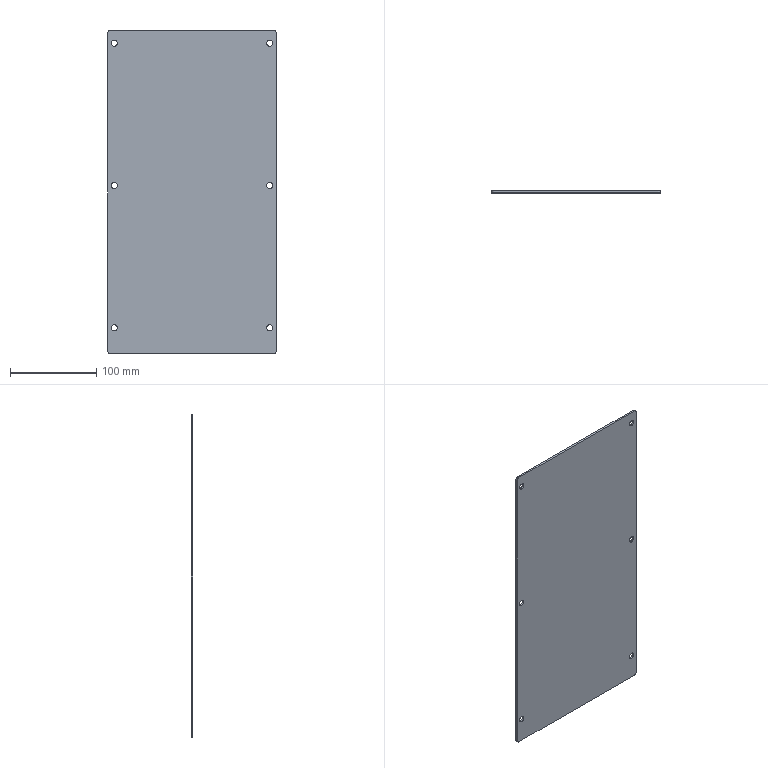Component | SolidWorks | CoverPlate4-1 | 1 solid | 22 faces | box 195 x 2 x 375 mm | volume 145773 mm3 | cylinder 16 | plane 6 | commonest cylinder face diameters 7 x12 6 x4 | material Plain Carbon Steel
build123d program:
from build123d import *

# Parameters (mm, degrees)
SKETCH1_W           = 375
SKETCH1_H           = 195
BOSS_EXTRUDE1_DEPTH = 2
SKETCH2_R           = 3.5
CUT_EXTRUDE1_DEPTH  = 2
FILLET1_R           = 3


with BuildPart() as part:
    # Sketch1 → Boss-Extrude1 (new body)
    with BuildSketch(Plane.XY):
        Rectangle(SKETCH1_W, SKETCH1_H)
    extrude(amount=BOSS_EXTRUDE1_DEPTH)

    # Sketch2 → Cut-Extrude1 (cut)
    with BuildSketch(Plane.XY.offset(2)):
        with Locations((-172.5, 90)):
            Circle(SKETCH2_R)
        with Locations((-7.5, 90)):
            Circle(SKETCH2_R)
        with Locations((-7.5, -90)):
            Circle(SKETCH2_R)
        with Locations((-172.5, -90)):
            Circle(SKETCH2_R)
        with Locations((157.5, 90)):
            Circle(SKETCH2_R)
        with Locations((157.5, -90)):
            Circle(SKETCH2_R)
    extrude(amount=-CUT_EXTRUDE1_DEPTH, mode=Mode.SUBTRACT)

    # Fillet1
    fillet1_edges = [part.edges().sort_by_distance(p)[0] for p in [
        (-187.5, 97.5, 1),
        (187.5, 97.5, 1),
        (187.5, -97.5, 1),
        (-187.5, -97.5, 1),
    ]]
    fillet(fillet1_edges, radius=FILLET1_R)


solid = part.part

# Placed as in the assembly
solid = solid.moved(Location((-47.166, -39.736, 10), (90, 0, -90)))
STEP:
#1=COLOUR_RGB('',0.7922,0.8196,0.9333);
#2=FILL_AREA_STYLE_COLOUR('',#1);
#3=FILL_AREA_STYLE('',(#2));
#4=SURFACE_STYLE_FILL_AREA(#3);
#5=SURFACE_SIDE_STYLE('',(#4));
#6=SURFACE_STYLE_USAGE(.BOTH.,#5);
#7=PRESENTATION_STYLE_ASSIGNMENT((#6));
#8=CARTESIAN_POINT('',(-5.4,-1.564,-5.669));
#9=VERTEX_POINT('',#8);
#10=CARTESIAN_POINT('',(-5.4,-1.564,-5.945));
#11=VERTEX_POINT('',#10);
#12=CARTESIAN_POINT('',(-5.4,-1.564,-5.807));
#13=DIRECTION('',(-0.,-1.,0.));
#14=DIRECTION('',(0.,0.,-1.));
#15=AXIS2_PLACEMENT_3D('',#12,#13,#14);
#16=CIRCLE('',#15,0.1378);
#17=EDGE_CURVE('',#9,#11,#16,.T.);
#18=ORIENTED_EDGE('',*,*,#17,.F.);
#19=CARTESIAN_POINT('',(-5.4,-1.643,-5.669));
#20=VERTEX_POINT('',#19);
#21=CARTESIAN_POINT('',(-5.4,-1.564,-5.669));
#22=DIRECTION('',(-0.,-1.,0.));
#23=VECTOR('',#22,39.37);
#24=LINE('',#21,#23);
#25=EDGE_CURVE('',#9,#20,#24,.T.);
#26=ORIENTED_EDGE('',*,*,#25,.T.);
#27=CARTESIAN_POINT('',(-5.4,-1.643,-5.945));
#28=VERTEX_POINT('',#27);
#29=CARTESIAN_POINT('',(-5.4,-1.643,-5.807));
#30=DIRECTION('',(-0.,-1.,0.));
#31=DIRECTION('',(0.,0.,-1.));
#32=AXIS2_PLACEMENT_3D('',#29,#30,#31);
#33=CIRCLE('',#32,0.1378);
#34=EDGE_CURVE('',#20,#28,#33,.T.);
#35=ORIENTED_EDGE('',*,*,#34,.T.);
#36=CARTESIAN_POINT('',(-5.4,-1.564,-5.945));
#37=DIRECTION('',(-0.,-1.,0.));
#38=VECTOR('',#37,39.37);
#39=LINE('',#36,#38);
#40=EDGE_CURVE('',#11,#28,#39,.T.);
#41=ORIENTED_EDGE('',*,*,#40,.F.);
#42=EDGE_LOOP('',(#18,#26,#35,#41));
#43=FACE_OUTER_BOUND('',#42,.T.);
#44=CARTESIAN_POINT('',(-5.4,-1.564,-5.807));
#45=DIRECTION('',(-0.,-1.,0.));
#46=DIRECTION('',(0.,0.,-1.));
#47=AXIS2_PLACEMENT_3D('',#44,#45,#46);
#48=CYLINDRICAL_SURFACE('',#47,0.1378);
#49=ADVANCED_FACE('',(#43),#48,.F.);
#50=CARTESIAN_POINT('',(1.686,-1.564,-5.669));
#51=VERTEX_POINT('',#50);
#52=CARTESIAN_POINT('',(1.686,-1.564,-5.945));
#53=VERTEX_POINT('',#52);
#54=CARTESIAN_POINT('',(1.686,-1.564,-5.807));
#55=DIRECTION('',(-0.,-1.,0.));
#56=DIRECTION('',(0.,0.,-1.));
#57=AXIS2_PLACEMENT_3D('',#54,#55,#56);
#58=CIRCLE('',#57,0.1378);
#59=EDGE_CURVE('',#51,#53,#58,.T.);
#60=ORIENTED_EDGE('',*,*,#59,.F.);
#61=CARTESIAN_POINT('',(1.686,-1.643,-5.669));
#62=VERTEX_POINT('',#61);
#63=CARTESIAN_POINT('',(1.686,-1.564,-5.669));
#64=DIRECTION('',(-0.,-1.,0.));
#65=VECTOR('',#64,39.37);
#66=LINE('',#63,#65);
#67=EDGE_CURVE('',#51,#62,#66,.T.);
#68=ORIENTED_EDGE('',*,*,#67,.T.);
#69=CARTESIAN_POINT('',(1.686,-1.643,-5.945));
#70=VERTEX_POINT('',#69);
#71=CARTESIAN_POINT('',(1.686,-1.643,-5.807));
#72=DIRECTION('',(-0.,-1.,0.));
#73=DIRECTION('',(0.,0.,-1.));
#74=AXIS2_PLACEMENT_3D('',#71,#72,#73);
#75=CIRCLE('',#74,0.1378);
#76=EDGE_CURVE('',#62,#70,#75,.T.);
#77=ORIENTED_EDGE('',*,*,#76,.T.);
#78=CARTESIAN_POINT('',(1.686,-1.564,-5.945));
#79=DIRECTION('',(-0.,-1.,0.));
#80=VECTOR('',#79,39.37);
#81=LINE('',#78,#80);
#82=EDGE_CURVE('',#53,#70,#81,.T.);
#83=ORIENTED_EDGE('',*,*,#82,.F.);
#84=EDGE_LOOP('',(#60,#68,#77,#83));
#85=FACE_OUTER_BOUND('',#84,.T.);
#86=CARTESIAN_POINT('',(1.686,-1.564,-5.807));
#87=DIRECTION('',(-0.,-1.,0.));
#88=DIRECTION('',(0.,0.,-1.));
#89=AXIS2_PLACEMENT_3D('',#86,#87,#88);
#90=CYLINDRICAL_SURFACE('',#89,0.1378);
#91=ADVANCED_FACE('',(#85),#90,.F.);
#92=CARTESIAN_POINT('',(-5.4,-1.564,7.323));
#93=VERTEX_POINT('',#92);
#94=CARTESIAN_POINT('',(-5.4,-1.564,7.047));
#95=VERTEX_POINT('',#94);
#96=CARTESIAN_POINT('',(-5.4,-1.564,7.185));
#97=DIRECTION('',(-0.,-1.,0.));
#98=DIRECTION('',(0.,0.,-1.));
#99=AXIS2_PLACEMENT_3D('',#96,#97,#98);
#100=CIRCLE('',#99,0.1378);
#101=EDGE_CURVE('',#93,#95,#100,.T.);
#102=ORIENTED_EDGE('',*,*,#101,.F.);
#103=CARTESIAN_POINT('',(-5.4,-1.643,7.323));
#104=VERTEX_POINT('',#103);
#105=CARTESIAN_POINT('',(-5.4,-1.564,7.323));
#106=DIRECTION('',(-0.,-1.,0.));
#107=VECTOR('',#106,39.37);
#108=LINE('',#105,#107);
#109=EDGE_CURVE('',#93,#104,#108,.T.);
#110=ORIENTED_EDGE('',*,*,#109,.T.);
#111=CARTESIAN_POINT('',(-5.4,-1.643,7.047));
#112=VERTEX_POINT('',#111);
#113=CARTESIAN_POINT('',(-5.4,-1.643,7.185));
#114=DIRECTION('',(-0.,-1.,0.));
#115=DIRECTION('',(0.,0.,-1.));
#116=AXIS2_PLACEMENT_3D('',#113,#114,#115);
#117=CIRCLE('',#116,0.1378);
#118=EDGE_CURVE('',#104,#112,#117,.T.);
#119=ORIENTED_EDGE('',*,*,#118,.T.);
#120=CARTESIAN_POINT('',(-5.4,-1.564,7.047));
#121=DIRECTION('',(-0.,-1.,0.));
#122=VECTOR('',#121,39.37);
#123=LINE('',#120,#122);
#124=EDGE_CURVE('',#95,#112,#123,.T.);
#125=ORIENTED_EDGE('',*,*,#124,.F.);
#126=EDGE_LOOP('',(#102,#110,#119,#125));
#127=FACE_OUTER_BOUND('',#126,.T.);
#128=CARTESIAN_POINT('',(-5.4,-1.564,7.185));
#129=DIRECTION('',(-0.,-1.,0.));
#130=DIRECTION('',(0.,0.,-1.));
#131=AXIS2_PLACEMENT_3D('',#128,#129,#130);
#132=CYLINDRICAL_SURFACE('',#131,0.1378);
#133=ADVANCED_FACE('',(#127),#132,.F.);
#134=CARTESIAN_POINT('',(-5.4,-1.564,0.8268));
#135=VERTEX_POINT('',#134);
#136=CARTESIAN_POINT('',(-5.4,-1.564,0.5512));
#137=VERTEX_POINT('',#136);
#138=CARTESIAN_POINT('',(-5.4,-1.564,0.689));
#139=DIRECTION('',(-0.,-1.,0.));
#140=DIRECTION('',(0.,0.,-1.));
#141=AXIS2_PLACEMENT_3D('',#138,#139,#140);
#142=CIRCLE('',#141,0.1378);
#143=EDGE_CURVE('',#135,#137,#142,.T.);
#144=ORIENTED_EDGE('',*,*,#143,.F.);
#145=CARTESIAN_POINT('',(-5.4,-1.643,0.8268));
#146=VERTEX_POINT('',#145);
#147=CARTESIAN_POINT('',(-5.4,-1.564,0.8268));
#148=DIRECTION('',(-0.,-1.,0.));
#149=VECTOR('',#148,39.37);
#150=LINE('',#147,#149);
#151=EDGE_CURVE('',#135,#146,#150,.T.);
#152=ORIENTED_EDGE('',*,*,#151,.T.);
#153=CARTESIAN_POINT('',(-5.4,-1.643,0.5512));
#154=VERTEX_POINT('',#153);
#155=CARTESIAN_POINT('',(-5.4,-1.643,0.689));
#156=DIRECTION('',(-0.,-1.,0.));
#157=DIRECTION('',(0.,0.,-1.));
#158=AXIS2_PLACEMENT_3D('',#155,#156,#157);
#159=CIRCLE('',#158,0.1378);
#160=EDGE_CURVE('',#146,#154,#159,.T.);
#161=ORIENTED_EDGE('',*,*,#160,.T.);
#162=CARTESIAN_POINT('',(-5.4,-1.564,0.5512));
#163=DIRECTION('',(-0.,-1.,0.));
#164=VECTOR('',#163,39.37);
#165=LINE('',#162,#164);
#166=EDGE_CURVE('',#137,#154,#165,.T.);
#167=ORIENTED_EDGE('',*,*,#166,.F.);
#168=EDGE_LOOP('',(#144,#152,#161,#167));
#169=FACE_OUTER_BOUND('',#168,.T.);
#170=CARTESIAN_POINT('',(-5.4,-1.564,0.689));
#171=DIRECTION('',(-0.,-1.,0.));
#172=DIRECTION('',(0.,0.,-1.));
#173=AXIS2_PLACEMENT_3D('',#170,#171,#172);
#174=CYLINDRICAL_SURFACE('',#173,0.1378);
#175=ADVANCED_FACE('',(#169),#174,.F.);
#176=CARTESIAN_POINT('',(1.686,-1.564,0.8268));
#177=VERTEX_POINT('',#176);
#178=CARTESIAN_POINT('',(1.686,-1.564,0.5512));
#179=VERTEX_POINT('',#178);
#180=CARTESIAN_POINT('',(1.686,-1.564,0.689));
#181=DIRECTION('',(-0.,-1.,0.));
#182=DIRECTION('',(0.,0.,-1.));
#183=AXIS2_PLACEMENT_3D('',#180,#181,#182);
#184=CIRCLE('',#183,0.1378);
#185=EDGE_CURVE('',#177,#179,#184,.T.);
#186=ORIENTED_EDGE('',*,*,#185,.F.);
#187=CARTESIAN_POINT('',(1.686,-1.643,0.8268));
#188=VERTEX_POINT('',#187);
#189=CARTESIAN_POINT('',(1.686,-1.564,0.8268));
#190=DIRECTION('',(-0.,-1.,0.));
#191=VECTOR('',#190,39.37);
#192=LINE('',#189,#191);
#193=EDGE_CURVE('',#177,#188,#192,.T.);
#194=ORIENTED_EDGE('',*,*,#193,.T.);
#195=CARTESIAN_POINT('',(1.686,-1.643,0.5512));
#196=VERTEX_POINT('',#195);
#197=CARTESIAN_POINT('',(1.686,-1.643,0.689));
#198=DIRECTION('',(-0.,-1.,0.));
#199=DIRECTION('',(0.,0.,-1.));
#200=AXIS2_PLACEMENT_3D('',#197,#198,#199);
#201=CIRCLE('',#200,0.1378);
#202=EDGE_CURVE('',#188,#196,#201,.T.);
#203=ORIENTED_EDGE('',*,*,#202,.T.);
#204=CARTESIAN_POINT('',(1.686,-1.564,0.5512));
#205=DIRECTION('',(-0.,-1.,0.));
#206=VECTOR('',#205,39.37);
#207=LINE('',#204,#206);
#208=EDGE_CURVE('',#179,#196,#207,.T.);
#209=ORIENTED_EDGE('',*,*,#208,.F.);
#210=EDGE_LOOP('',(#186,#194,#203,#209));
#211=FACE_OUTER_BOUND('',#210,.T.);
#212=CARTESIAN_POINT('',(1.686,-1.564,0.689));
#213=DIRECTION('',(-0.,-1.,0.));
#214=DIRECTION('',(0.,0.,-1.));
#215=AXIS2_PLACEMENT_3D('',#212,#213,#214);
#216=CYLINDRICAL_SURFACE('',#215,0.1378);
#217=ADVANCED_FACE('',(#211),#216,.F.);
#218=CARTESIAN_POINT('',(1.686,-1.564,7.323));
#219=VERTEX_POINT('',#218);
#220=CARTESIAN_POINT('',(1.686,-1.564,7.047));
#221=VERTEX_POINT('',#220);
#222=CARTESIAN_POINT('',(1.686,-1.564,7.185));
#223=DIRECTION('',(-0.,-1.,0.));
#224=DIRECTION('',(0.,0.,-1.));
#225=AXIS2_PLACEMENT_3D('',#222,#223,#224);
#226=CIRCLE('',#225,0.1378);
#227=EDGE_CURVE('',#219,#221,#226,.T.);
#228=ORIENTED_EDGE('',*,*,#227,.F.);
#229=CARTESIAN_POINT('',(1.686,-1.643,7.323));
#230=VERTEX_POINT('',#229);
#231=CARTESIAN_POINT('',(1.686,-1.564,7.323));
#232=DIRECTION('',(-0.,-1.,0.));
#233=VECTOR('',#232,39.37);
#234=LINE('',#231,#233);
#235=EDGE_CURVE('',#219,#230,#234,.T.);
#236=ORIENTED_EDGE('',*,*,#235,.T.);
#237=CARTESIAN_POINT('',(1.686,-1.643,7.047));
#238=VERTEX_POINT('',#237);
#239=CARTESIAN_POINT('',(1.686,-1.643,7.185));
#240=DIRECTION('',(-0.,-1.,0.));
#241=DIRECTION('',(0.,0.,-1.));
#242=AXIS2_PLACEMENT_3D('',#239,#240,#241);
#243=CIRCLE('',#242,0.1378);
#244=EDGE_CURVE('',#230,#238,#243,.T.);
#245=ORIENTED_EDGE('',*,*,#244,.T.);
#246=CARTESIAN_POINT('',(1.686,-1.564,7.047));
#247=DIRECTION('',(-0.,-1.,0.));
#248=VECTOR('',#247,39.37);
#249=LINE('',#246,#248);
#250=EDGE_CURVE('',#221,#238,#249,.T.);
#251=ORIENTED_EDGE('',*,*,#250,.F.);
#252=EDGE_LOOP('',(#228,#236,#245,#251));
#253=FACE_OUTER_BOUND('',#252,.T.);
#254=CARTESIAN_POINT('',(1.686,-1.564,7.185));
#255=DIRECTION('',(-0.,-1.,0.));
#256=DIRECTION('',(0.,0.,-1.));
#257=AXIS2_PLACEMENT_3D('',#254,#255,#256);
#258=CYLINDRICAL_SURFACE('',#257,0.1378);
#259=ADVANCED_FACE('',(#253),#258,.F.);
#260=CARTESIAN_POINT('',(1.864,-1.564,7.776));
#261=VERTEX_POINT('',#260);
#262=CARTESIAN_POINT('',(-5.577,-1.564,7.776));
#263=VERTEX_POINT('',#262);
#264=CARTESIAN_POINT('',(1.982,-1.564,7.776));
#265=DIRECTION('',(-1.,0.,0.));
#266=VECTOR('',#265,39.37);
#267=LINE('',#264,#266);
#268=EDGE_CURVE('',#261,#263,#267,.T.);
#269=ORIENTED_EDGE('',*,*,#268,.T.);
#270=CARTESIAN_POINT('',(-5.577,-1.643,7.776));
#271=VERTEX_POINT('',#270);
#272=CARTESIAN_POINT('',(-5.577,-1.643,7.776));
#273=DIRECTION('',(-0.,-1.,0.));
#274=VECTOR('',#273,39.37);
#275=LINE('',#272,#274);
#276=EDGE_CURVE('',#263,#271,#275,.T.);
#277=ORIENTED_EDGE('',*,*,#276,.T.);
#278=CARTESIAN_POINT('',(1.864,-1.643,7.776));
#279=VERTEX_POINT('',#278);
#280=CARTESIAN_POINT('',(1.982,-1.643,7.776));
#281=DIRECTION('',(-1.,0.,0.));
#282=VECTOR('',#281,39.37);
#283=LINE('',#280,#282);
#284=EDGE_CURVE('',#279,#271,#283,.T.);
#285=ORIENTED_EDGE('',*,*,#284,.F.);
#286=CARTESIAN_POINT('',(1.864,-1.643,7.776));
#287=DIRECTION('',(0.,1.,-0.));
#288=VECTOR('',#287,39.37);
#289=LINE('',#286,#288);
#290=EDGE_CURVE('',#279,#261,#289,.T.);
#291=ORIENTED_EDGE('',*,*,#290,.T.);
#292=EDGE_LOOP('',(#269,#277,#285,#291));
#293=FACE_OUTER_BOUND('',#292,.T.);
#294=CARTESIAN_POINT('',(1.982,-1.643,7.776));
#295=DIRECTION('',(-0.,-0.,-1.));
#296=DIRECTION('',(0.,1.,-0.));
#297=AXIS2_PLACEMENT_3D('',#294,#295,#296);
#298=PLANE('',#297);
#299=ADVANCED_FACE('',(#293),#298,.F.);
#300=CARTESIAN_POINT('',(-5.696,-1.564,7.657));
#301=VERTEX_POINT('',#300);
#302=CARTESIAN_POINT('',(-5.696,-1.564,-6.87));
#303=VERTEX_POINT('',#302);
#304=CARTESIAN_POINT('',(-5.696,-1.564,7.776));
#305=DIRECTION('',(-0.,-0.,-1.));
#306=VECTOR('',#305,39.37);
#307=LINE('',#304,#306);
#308=EDGE_CURVE('',#301,#303,#307,.T.);
#309=ORIENTED_EDGE('',*,*,#308,.T.);
#310=CARTESIAN_POINT('',(-5.696,-1.643,-6.87));
#311=VERTEX_POINT('',#310);
#312=CARTESIAN_POINT('',(-5.696,-1.643,-6.87));
#313=DIRECTION('',(-0.,-1.,0.));
#314=VECTOR('',#313,39.37);
#315=LINE('',#312,#314);
#316=EDGE_CURVE('',#303,#311,#315,.T.);
#317=ORIENTED_EDGE('',*,*,#316,.T.);
#318=CARTESIAN_POINT('',(-5.696,-1.643,7.657));
#319=VERTEX_POINT('',#318);
#320=CARTESIAN_POINT('',(-5.696,-1.643,7.776));
#321=DIRECTION('',(-0.,-0.,-1.));
#322=VECTOR('',#321,39.37);
#323=LINE('',#320,#322);
#324=EDGE_CURVE('',#319,#311,#323,.T.);
#325=ORIENTED_EDGE('',*,*,#324,.F.);
#326=CARTESIAN_POINT('',(-5.696,-1.643,7.657));
#327=DIRECTION('',(0.,1.,-0.));
#328=VECTOR('',#327,39.37);
#329=LINE('',#326,#328);
#330=EDGE_CURVE('',#319,#301,#329,.T.);
#331=ORIENTED_EDGE('',*,*,#330,.T.);
#332=EDGE_LOOP('',(#309,#317,#325,#331));
#333=FACE_OUTER_BOUND('',#332,.T.);
#334=CARTESIAN_POINT('',(-5.696,-1.643,7.776));
#335=DIRECTION('',(1.,-0.,-0.));
#336=DIRECTION('',(-0.,-1.,0.));
#337=AXIS2_PLACEMENT_3D('',#334,#335,#336);
#338=PLANE('',#337);
#339=ADVANCED_FACE('',(#333),#338,.F.);
#340=CARTESIAN_POINT('',(-5.577,-1.643,-6.988));
#341=VERTEX_POINT('',#340);
#342=CARTESIAN_POINT('',(1.864,-1.643,-6.988));
#343=VERTEX_POINT('',#342);
#344=CARTESIAN_POINT('',(1.982,-1.643,-6.988));
#345=DIRECTION('',(1.,-0.,0.));
#346=VECTOR('',#345,39.37);
#347=LINE('',#344,#346);
#348=EDGE_CURVE('',#341,#343,#347,.T.);
#349=ORIENTED_EDGE('',*,*,#348,.F.);
#350=CARTESIAN_POINT('',(-5.577,-1.564,-6.988));
#351=VERTEX_POINT('',#350);
#352=CARTESIAN_POINT('',(-5.577,-1.643,-6.988));
#353=DIRECTION('',(0.,1.,-0.));
#354=VECTOR('',#353,39.37);
#355=LINE('',#352,#354);
#356=EDGE_CURVE('',#341,#351,#355,.T.);
#357=ORIENTED_EDGE('',*,*,#356,.T.);
#358=CARTESIAN_POINT('',(1.864,-1.564,-6.988));
#359=VERTEX_POINT('',#358);
#360=CARTESIAN_POINT('',(1.982,-1.564,-6.988));
#361=DIRECTION('',(1.,-0.,0.));
#362=VECTOR('',#361,39.37);
#363=LINE('',#360,#362);
#364=EDGE_CURVE('',#351,#359,#363,.T.);
#365=ORIENTED_EDGE('',*,*,#364,.T.);
#366=CARTESIAN_POINT('',(1.864,-1.643,-6.988));
#367=DIRECTION('',(-0.,-1.,0.));
#368=VECTOR('',#367,39.37);
#369=LINE('',#366,#368);
#370=EDGE_CURVE('',#359,#343,#369,.T.);
#371=ORIENTED_EDGE('',*,*,#370,.T.);
#372=EDGE_LOOP('',(#349,#357,#365,#371));
#373=FACE_OUTER_BOUND('',#372,.T.);
#374=CARTESIAN_POINT('',(1.982,-1.643,-6.988));
#375=DIRECTION('',(-0.,0.,1.));
#376=DIRECTION('',(-1.,0.,-0.));
#377=AXIS2_PLACEMENT_3D('',#374,#375,#376);
#378=PLANE('',#377);
#379=ADVANCED_FACE('',(#373),#378,.F.);
#380=CARTESIAN_POINT('',(1.982,-1.643,-6.87));
#381=VERTEX_POINT('',#380);
#382=CARTESIAN_POINT('',(1.982,-1.643,7.657));
#383=VERTEX_POINT('',#382);
#384=CARTESIAN_POINT('',(1.982,-1.643,7.776));
#385=DIRECTION('',(0.,0.,1.));
#386=VECTOR('',#385,39.37);
#387=LINE('',#384,#386);
#388=EDGE_CURVE('',#381,#383,#387,.T.);
#389=ORIENTED_EDGE('',*,*,#388,.F.);
#390=CARTESIAN_POINT('',(1.982,-1.564,-6.87));
#391=VERTEX_POINT('',#390);
#392=CARTESIAN_POINT('',(1.982,-1.643,-6.87));
#393=DIRECTION('',(0.,1.,-0.));
#394=VECTOR('',#393,39.37);
#395=LINE('',#392,#394);
#396=EDGE_CURVE('',#381,#391,#395,.T.);
#397=ORIENTED_EDGE('',*,*,#396,.T.);
#398=CARTESIAN_POINT('',(1.982,-1.564,7.657));
#399=VERTEX_POINT('',#398);
#400=CARTESIAN_POINT('',(1.982,-1.564,7.776));
#401=DIRECTION('',(0.,0.,1.));
#402=VECTOR('',#401,39.37);
#403=LINE('',#400,#402);
#404=EDGE_CURVE('',#391,#399,#403,.T.);
#405=ORIENTED_EDGE('',*,*,#404,.T.);
#406=CARTESIAN_POINT('',(1.982,-1.643,7.657));
#407=DIRECTION('',(-0.,-1.,0.));
#408=VECTOR('',#407,39.37);
#409=LINE('',#406,#408);
#410=EDGE_CURVE('',#399,#383,#409,.T.);
#411=ORIENTED_EDGE('',*,*,#410,.T.);
#412=EDGE_LOOP('',(#389,#397,#405,#411));
#413=FACE_OUTER_BOUND('',#412,.T.);
#414=CARTESIAN_POINT('',(1.982,-1.643,7.776));
#415=DIRECTION('',(-1.,0.,0.));
#416=DIRECTION('',(-0.,-0.,-1.));
#417=AXIS2_PLACEMENT_3D('',#414,#415,#416);
#418=PLANE('',#417);
#419=ADVANCED_FACE('',(#413),#418,.F.);
#420=CARTESIAN_POINT('',(-5.4,-1.643,-5.807));
#421=DIRECTION('',(-0.,-1.,0.));
#422=DIRECTION('',(0.,0.,-1.));
#423=AXIS2_PLACEMENT_3D('',#420,#421,#422);
#424=CIRCLE('',#423,0.1378);
#425=EDGE_CURVE('',#28,#20,#424,.T.);
#426=ORIENTED_EDGE('',*,*,#425,.F.);
#427=ORIENTED_EDGE('',*,*,#34,.F.);
#428=EDGE_LOOP('',(#426,#427));
#429=FACE_BOUND('',#428,.T.);
#430=CARTESIAN_POINT('',(1.686,-1.643,-5.807));
#431=DIRECTION('',(-0.,-1.,0.));
#432=DIRECTION('',(0.,0.,-1.));
#433=AXIS2_PLACEMENT_3D('',#430,#431,#432);
#434=CIRCLE('',#433,0.1378);
#435=EDGE_CURVE('',#70,#62,#434,.T.);
#436=ORIENTED_EDGE('',*,*,#435,.F.);
#437=ORIENTED_EDGE('',*,*,#76,.F.);
#438=EDGE_LOOP('',(#436,#437));
#439=FACE_BOUND('',#438,.T.);
#440=CARTESIAN_POINT('',(-5.4,-1.643,7.185));
#441=DIRECTION('',(-0.,-1.,0.));
#442=DIRECTION('',(0.,0.,-1.));
#443=AXIS2_PLACEMENT_3D('',#440,#441,#442);
#444=CIRCLE('',#443,0.1378);
#445=EDGE_CURVE('',#112,#104,#444,.T.);
#446=ORIENTED_EDGE('',*,*,#445,.F.);
#447=ORIENTED_EDGE('',*,*,#118,.F.);
#448=EDGE_LOOP('',(#446,#447));
#449=FACE_BOUND('',#448,.T.);
#450=CARTESIAN_POINT('',(-5.4,-1.643,0.689));
#451=DIRECTION('',(-0.,-1.,0.));
#452=DIRECTION('',(0.,0.,-1.));
#453=AXIS2_PLACEMENT_3D('',#450,#451,#452);
#454=CIRCLE('',#453,0.1378);
#455=EDGE_CURVE('',#154,#146,#454,.T.);
#456=ORIENTED_EDGE('',*,*,#455,.F.);
#457=ORIENTED_EDGE('',*,*,#160,.F.);
#458=EDGE_LOOP('',(#456,#457));
#459=FACE_BOUND('',#458,.T.);
#460=CARTESIAN_POINT('',(1.686,-1.643,0.689));
#461=DIRECTION('',(-0.,-1.,0.));
#462=DIRECTION('',(0.,0.,-1.));
#463=AXIS2_PLACEMENT_3D('',#460,#461,#462);
#464=CIRCLE('',#463,0.1378);
#465=EDGE_CURVE('',#196,#188,#464,.T.);
#466=ORIENTED_EDGE('',*,*,#465,.F.);
#467=ORIENTED_EDGE('',*,*,#202,.F.);
#468=EDGE_LOOP('',(#466,#467));
#469=FACE_BOUND('',#468,.T.);
#470=CARTESIAN_POINT('',(1.686,-1.643,7.185));
#471=DIRECTION('',(-0.,-1.,0.));
#472=DIRECTION('',(0.,0.,-1.));
#473=AXIS2_PLACEMENT_3D('',#470,#471,#472);
#474=CIRCLE('',#473,0.1378);
#475=EDGE_CURVE('',#238,#230,#474,.T.);
#476=ORIENTED_EDGE('',*,*,#475,.F.);
#477=ORIENTED_EDGE('',*,*,#244,.F.);
#478=EDGE_LOOP('',(#476,#477));
#479=FACE_BOUND('',#478,.T.);
#480=ORIENTED_EDGE('',*,*,#324,.T.);
#481=CARTESIAN_POINT('',(-5.577,-1.643,-6.87));
#482=DIRECTION('',(-0.,-1.,0.));
#483=DIRECTION('',(0.,0.,-1.));
#484=AXIS2_PLACEMENT_3D('',#481,#482,#483);
#485=CIRCLE('',#484,0.1181);
#486=EDGE_CURVE('',#311,#341,#485,.T.);
#487=ORIENTED_EDGE('',*,*,#486,.T.);
#488=ORIENTED_EDGE('',*,*,#348,.T.);
#489=CARTESIAN_POINT('',(1.864,-1.643,-6.87));
#490=DIRECTION('',(-0.,-1.,0.));
#491=DIRECTION('',(0.,0.,-1.));
#492=AXIS2_PLACEMENT_3D('',#489,#490,#491);
#493=CIRCLE('',#492,0.1181);
#494=EDGE_CURVE('',#343,#381,#493,.T.);
#495=ORIENTED_EDGE('',*,*,#494,.T.);
#496=ORIENTED_EDGE('',*,*,#388,.T.);
#497=CARTESIAN_POINT('',(1.864,-1.643,7.657));
#498=DIRECTION('',(-0.,-1.,0.));
#499=DIRECTION('',(0.,0.,-1.));
#500=AXIS2_PLACEMENT_3D('',#497,#498,#499);
#501=CIRCLE('',#500,0.1181);
#502=EDGE_CURVE('',#383,#279,#501,.T.);
#503=ORIENTED_EDGE('',*,*,#502,.T.);
#504=ORIENTED_EDGE('',*,*,#284,.T.);
#505=CARTESIAN_POINT('',(-5.577,-1.643,7.657));
#506=DIRECTION('',(-0.,-1.,0.));
#507=DIRECTION('',(0.,0.,-1.));
#508=AXIS2_PLACEMENT_3D('',#505,#506,#507);
#509=CIRCLE('',#508,0.1181);
#510=EDGE_CURVE('',#271,#319,#509,.T.);
#511=ORIENTED_EDGE('',*,*,#510,.T.);
#512=EDGE_LOOP('',(#480,#487,#488,#495,#496,#503,#504,#511));
#513=FACE_OUTER_BOUND('',#512,.T.);
#514=CARTESIAN_POINT('',(-1.857,-1.643,0.3937));
#515=DIRECTION('',(-0.,-1.,0.));
#516=DIRECTION('',(-0.,-0.,-1.));
#517=AXIS2_PLACEMENT_3D('',#514,#515,#516);
#518=PLANE('',#517);
#519=ADVANCED_FACE('',(#429,#439,#449,#459,#469,#479,#513),#518,.T.);
#520=CARTESIAN_POINT('',(-5.4,-1.564,-5.807));
#521=DIRECTION('',(-0.,-1.,0.));
#522=DIRECTION('',(0.,0.,-1.));
#523=AXIS2_PLACEMENT_3D('',#520,#521,#522);
#524=CIRCLE('',#523,0.1378);
#525=EDGE_CURVE('',#11,#9,#524,.T.);
#526=ORIENTED_EDGE('',*,*,#525,.T.);
#527=ORIENTED_EDGE('',*,*,#17,.T.);
#528=EDGE_LOOP('',(#526,#527));
#529=FACE_BOUND('',#528,.T.);
#530=CARTESIAN_POINT('',(1.686,-1.564,-5.807));
#531=DIRECTION('',(-0.,-1.,0.));
#532=DIRECTION('',(0.,0.,-1.));
#533=AXIS2_PLACEMENT_3D('',#530,#531,#532);
#534=CIRCLE('',#533,0.1378);
#535=EDGE_CURVE('',#53,#51,#534,.T.);
#536=ORIENTED_EDGE('',*,*,#535,.T.);
#537=ORIENTED_EDGE('',*,*,#59,.T.);
#538=EDGE_LOOP('',(#536,#537));
#539=FACE_BOUND('',#538,.T.);
#540=CARTESIAN_POINT('',(-5.4,-1.564,7.185));
#541=DIRECTION('',(-0.,-1.,0.));
#542=DIRECTION('',(0.,0.,-1.));
#543=AXIS2_PLACEMENT_3D('',#540,#541,#542);
#544=CIRCLE('',#543,0.1378);
#545=EDGE_CURVE('',#95,#93,#544,.T.);
#546=ORIENTED_EDGE('',*,*,#545,.T.);
#547=ORIENTED_EDGE('',*,*,#101,.T.);
#548=EDGE_LOOP('',(#546,#547));
#549=FACE_BOUND('',#548,.T.);
#550=CARTESIAN_POINT('',(-5.4,-1.564,0.689));
#551=DIRECTION('',(-0.,-1.,0.));
#552=DIRECTION('',(0.,0.,-1.));
#553=AXIS2_PLACEMENT_3D('',#550,#551,#552);
#554=CIRCLE('',#553,0.1378);
#555=EDGE_CURVE('',#137,#135,#554,.T.);
#556=ORIENTED_EDGE('',*,*,#555,.T.);
#557=ORIENTED_EDGE('',*,*,#143,.T.);
#558=EDGE_LOOP('',(#556,#557));
#559=FACE_BOUND('',#558,.T.);
#560=CARTESIAN_POINT('',(1.686,-1.564,0.689));
#561=DIRECTION('',(-0.,-1.,0.));
#562=DIRECTION('',(0.,0.,-1.));
#563=AXIS2_PLACEMENT_3D('',#560,#561,#562);
#564=CIRCLE('',#563,0.1378);
#565=EDGE_CURVE('',#179,#177,#564,.T.);
#566=ORIENTED_EDGE('',*,*,#565,.T.);
#567=ORIENTED_EDGE('',*,*,#185,.T.);
#568=EDGE_LOOP('',(#566,#567));
#569=FACE_BOUND('',#568,.T.);
#570=CARTESIAN_POINT('',(1.686,-1.564,7.185));
#571=DIRECTION('',(-0.,-1.,0.));
#572=DIRECTION('',(0.,0.,-1.));
#573=AXIS2_PLACEMENT_3D('',#570,#571,#572);
#574=CIRCLE('',#573,0.1378);
#575=EDGE_CURVE('',#221,#219,#574,.T.);
#576=ORIENTED_EDGE('',*,*,#575,.T.);
#577=ORIENTED_EDGE('',*,*,#227,.T.);
#578=EDGE_LOOP('',(#576,#577));
#579=FACE_BOUND('',#578,.T.);
#580=ORIENTED_EDGE('',*,*,#364,.F.);
#581=CARTESIAN_POINT('',(-5.577,-1.564,-6.87));
#582=DIRECTION('',(0.,1.,-0.));
#583=DIRECTION('',(0.,0.,-1.));
#584=AXIS2_PLACEMENT_3D('',#581,#582,#583);
#585=CIRCLE('',#584,0.1181);
#586=EDGE_CURVE('',#351,#303,#585,.T.);
#587=ORIENTED_EDGE('',*,*,#586,.T.);
#588=ORIENTED_EDGE('',*,*,#308,.F.);
#589=CARTESIAN_POINT('',(-5.577,-1.564,7.657));
#590=DIRECTION('',(0.,1.,-0.));
#591=DIRECTION('',(0.,0.,-1.));
#592=AXIS2_PLACEMENT_3D('',#589,#590,#591);
#593=CIRCLE('',#592,0.1181);
#594=EDGE_CURVE('',#301,#263,#593,.T.);
#595=ORIENTED_EDGE('',*,*,#594,.T.);
#596=ORIENTED_EDGE('',*,*,#268,.F.);
#597=CARTESIAN_POINT('',(1.864,-1.564,7.657));
#598=DIRECTION('',(0.,1.,-0.));
#599=DIRECTION('',(0.,0.,-1.));
#600=AXIS2_PLACEMENT_3D('',#597,#598,#599);
#601=CIRCLE('',#600,0.1181);
#602=EDGE_CURVE('',#261,#399,#601,.T.);
#603=ORIENTED_EDGE('',*,*,#602,.T.);
#604=ORIENTED_EDGE('',*,*,#404,.F.);
#605=CARTESIAN_POINT('',(1.864,-1.564,-6.87));
#606=DIRECTION('',(0.,1.,-0.));
#607=DIRECTION('',(0.,0.,-1.));
#608=AXIS2_PLACEMENT_3D('',#605,#606,#607);
#609=CIRCLE('',#608,0.1181);
#610=EDGE_CURVE('',#391,#359,#609,.T.);
#611=ORIENTED_EDGE('',*,*,#610,.T.);
#612=EDGE_LOOP('',(#580,#587,#588,#595,#596,#603,#604,#611));
#613=FACE_OUTER_BOUND('',#612,.T.);
#614=CARTESIAN_POINT('',(-1.857,-1.564,0.3937));
#615=DIRECTION('',(-0.,-1.,0.));
#616=DIRECTION('',(-0.,-0.,-1.));
#617=AXIS2_PLACEMENT_3D('',#614,#615,#616);
#618=PLANE('',#617);
#619=ADVANCED_FACE('',(#529,#539,#549,#559,#569,#579,#613),#618,.F.);
#620=ORIENTED_EDGE('',*,*,#235,.F.);
#621=ORIENTED_EDGE('',*,*,#575,.F.);
#622=ORIENTED_EDGE('',*,*,#250,.T.);
#623=ORIENTED_EDGE('',*,*,#475,.T.);
#624=EDGE_LOOP('',(#620,#621,#622,#623));
#625=FACE_OUTER_BOUND('',#624,.T.);
#626=CARTESIAN_POINT('',(1.686,-1.564,7.185));
#627=DIRECTION('',(-0.,-1.,0.));
#628=DIRECTION('',(0.,0.,-1.));
#629=AXIS2_PLACEMENT_3D('',#626,#627,#628);
#630=CYLINDRICAL_SURFACE('',#629,0.1378);
#631=ADVANCED_FACE('',(#625),#630,.F.);
#632=ORIENTED_EDGE('',*,*,#193,.F.);
#633=ORIENTED_EDGE('',*,*,#565,.F.);
#634=ORIENTED_EDGE('',*,*,#208,.T.);
#635=ORIENTED_EDGE('',*,*,#465,.T.);
#636=EDGE_LOOP('',(#632,#633,#634,#635));
#637=FACE_OUTER_BOUND('',#636,.T.);
#638=CARTESIAN_POINT('',(1.686,-1.564,0.689));
#639=DIRECTION('',(-0.,-1.,0.));
#640=DIRECTION('',(0.,0.,-1.));
#641=AXIS2_PLACEMENT_3D('',#638,#639,#640);
#642=CYLINDRICAL_SURFACE('',#641,0.1378);
#643=ADVANCED_FACE('',(#637),#642,.F.);
#644=ORIENTED_EDGE('',*,*,#151,.F.);
#645=ORIENTED_EDGE('',*,*,#555,.F.);
#646=ORIENTED_EDGE('',*,*,#166,.T.);
#647=ORIENTED_EDGE('',*,*,#455,.T.);
#648=EDGE_LOOP('',(#644,#645,#646,#647));
#649=FACE_OUTER_BOUND('',#648,.T.);
#650=CARTESIAN_POINT('',(-5.4,-1.564,0.689));
#651=DIRECTION('',(-0.,-1.,0.));
#652=DIRECTION('',(0.,0.,-1.));
#653=AXIS2_PLACEMENT_3D('',#650,#651,#652);
#654=CYLINDRICAL_SURFACE('',#653,0.1378);
#655=ADVANCED_FACE('',(#649),#654,.F.);
#656=ORIENTED_EDGE('',*,*,#109,.F.);
#657=ORIENTED_EDGE('',*,*,#545,.F.);
#658=ORIENTED_EDGE('',*,*,#124,.T.);
#659=ORIENTED_EDGE('',*,*,#445,.T.);
#660=EDGE_LOOP('',(#656,#657,#658,#659));
#661=FACE_OUTER_BOUND('',#660,.T.);
#662=CARTESIAN_POINT('',(-5.4,-1.564,7.185));
#663=DIRECTION('',(-0.,-1.,0.));
#664=DIRECTION('',(0.,0.,-1.));
#665=AXIS2_PLACEMENT_3D('',#662,#663,#664);
#666=CYLINDRICAL_SURFACE('',#665,0.1378);
#667=ADVANCED_FACE('',(#661),#666,.F.);
#668=ORIENTED_EDGE('',*,*,#67,.F.);
#669=ORIENTED_EDGE('',*,*,#535,.F.);
#670=ORIENTED_EDGE('',*,*,#82,.T.);
#671=ORIENTED_EDGE('',*,*,#435,.T.);
#672=EDGE_LOOP('',(#668,#669,#670,#671));
#673=FACE_OUTER_BOUND('',#672,.T.);
#674=CARTESIAN_POINT('',(1.686,-1.564,-5.807));
#675=DIRECTION('',(-0.,-1.,0.));
#676=DIRECTION('',(0.,0.,-1.));
#677=AXIS2_PLACEMENT_3D('',#674,#675,#676);
#678=CYLINDRICAL_SURFACE('',#677,0.1378);
#679=ADVANCED_FACE('',(#673),#678,.F.);
#680=ORIENTED_EDGE('',*,*,#25,.F.);
#681=ORIENTED_EDGE('',*,*,#525,.F.);
#682=ORIENTED_EDGE('',*,*,#40,.T.);
#683=ORIENTED_EDGE('',*,*,#425,.T.);
#684=EDGE_LOOP('',(#680,#681,#682,#683));
#685=FACE_OUTER_BOUND('',#684,.T.);
#686=CARTESIAN_POINT('',(-5.4,-1.564,-5.807));
#687=DIRECTION('',(-0.,-1.,0.));
#688=DIRECTION('',(0.,0.,-1.));
#689=AXIS2_PLACEMENT_3D('',#686,#687,#688);
#690=CYLINDRICAL_SURFACE('',#689,0.1378);
#691=ADVANCED_FACE('',(#685),#690,.F.);
#692=ORIENTED_EDGE('',*,*,#486,.F.);
#693=ORIENTED_EDGE('',*,*,#316,.F.);
#694=ORIENTED_EDGE('',*,*,#586,.F.);
#695=ORIENTED_EDGE('',*,*,#356,.F.);
#696=EDGE_LOOP('',(#692,#693,#694,#695));
#697=FACE_OUTER_BOUND('',#696,.T.);
#698=CARTESIAN_POINT('',(-5.577,-1.643,-6.87));
#699=DIRECTION('',(0.,1.,-0.));
#700=DIRECTION('',(0.,0.,1.));
#701=AXIS2_PLACEMENT_3D('',#698,#699,#700);
#702=CYLINDRICAL_SURFACE('',#701,0.1181);
#703=ADVANCED_FACE('',(#697),#702,.T.);
#704=ORIENTED_EDGE('',*,*,#494,.F.);
#705=ORIENTED_EDGE('',*,*,#370,.F.);
#706=ORIENTED_EDGE('',*,*,#610,.F.);
#707=ORIENTED_EDGE('',*,*,#396,.F.);
#708=EDGE_LOOP('',(#704,#705,#706,#707));
#709=FACE_OUTER_BOUND('',#708,.T.);
#710=CARTESIAN_POINT('',(1.864,-1.643,-6.87));
#711=DIRECTION('',(0.,1.,-0.));
#712=DIRECTION('',(0.,0.,1.));
#713=AXIS2_PLACEMENT_3D('',#710,#711,#712);
#714=CYLINDRICAL_SURFACE('',#713,0.1181);
#715=ADVANCED_FACE('',(#709),#714,.T.);
#716=ORIENTED_EDGE('',*,*,#510,.F.);
#717=ORIENTED_EDGE('',*,*,#276,.F.);
#718=ORIENTED_EDGE('',*,*,#594,.F.);
#719=ORIENTED_EDGE('',*,*,#330,.F.);
#720=EDGE_LOOP('',(#716,#717,#718,#719));
#721=FACE_OUTER_BOUND('',#720,.T.);
#722=CARTESIAN_POINT('',(-5.577,-1.643,7.657));
#723=DIRECTION('',(0.,1.,-0.));
#724=DIRECTION('',(0.,0.,1.));
#725=AXIS2_PLACEMENT_3D('',#722,#723,#724);
#726=CYLINDRICAL_SURFACE('',#725,0.1181);
#727=ADVANCED_FACE('',(#721),#726,.T.);
#728=ORIENTED_EDGE('',*,*,#502,.F.);
#729=ORIENTED_EDGE('',*,*,#410,.F.);
#730=ORIENTED_EDGE('',*,*,#602,.F.);
#731=ORIENTED_EDGE('',*,*,#290,.F.);
#732=EDGE_LOOP('',(#728,#729,#730,#731));
#733=FACE_OUTER_BOUND('',#732,.T.);
#734=CARTESIAN_POINT('',(1.864,-1.643,7.657));
#735=DIRECTION('',(0.,1.,-0.));
#736=DIRECTION('',(0.,0.,1.));
#737=AXIS2_PLACEMENT_3D('',#734,#735,#736);
#738=CYLINDRICAL_SURFACE('',#737,0.1181);
#739=ADVANCED_FACE('',(#733),#738,.T.);
#740=CLOSED_SHELL('',(#49,#91,#133,#175,#217,#259,#299,#339,#379,#419,#519,#619,#631,#643,#655,#667,#679,#691,#703,#715,#727,#739));
#741=MANIFOLD_SOLID_BREP('',#740);
#742=STYLED_ITEM('',(#7),#741);
#743=PRESENTATION_LAYER_ASSIGNMENT('','',(#742));
#744=(LENGTH_UNIT()NAMED_UNIT(*)SI_UNIT($,.METRE.));
#745=LENGTH_MEASURE_WITH_UNIT(LENGTH_MEASURE(0.0254),#744);
#746=DIMENSIONAL_EXPONENTS(1.,0.,0.,0.,0.,0.,0.);
#747=(CONVERSION_BASED_UNIT('',#745)LENGTH_UNIT()NAMED_UNIT(#746));
#748=UNCERTAINTY_MEASURE_WITH_UNIT(LENGTH_MEASURE(0.00001),#747,'','');
#749=(NAMED_UNIT(*)PLANE_ANGLE_UNIT()SI_UNIT($,.RADIAN.));
#750=(NAMED_UNIT(*)SI_UNIT($,.STERADIAN.)SOLID_ANGLE_UNIT());
#751=(GEOMETRIC_REPRESENTATION_CONTEXT(3)GLOBAL_UNCERTAINTY_ASSIGNED_CONTEXT((#748))GLOBAL_UNIT_ASSIGNED_CONTEXT((#747,#749,#750))REPRESENTATION_CONTEXT('',''));
#752=MECHANICAL_DESIGN_GEOMETRIC_PRESENTATION_REPRESENTATION('',(#742),#751);
#753=CARTESIAN_POINT('',(0.,0.,0.));
#754=DIRECTION('',(0.,0.,1.));
#755=DIRECTION('',(1.,0.,0.));
#756=AXIS2_PLACEMENT_3D('',#753,#754,#755);
#757=(LENGTH_UNIT()NAMED_UNIT(*)SI_UNIT($,.METRE.));
#758=LENGTH_MEASURE_WITH_UNIT(LENGTH_MEASURE(0.0254),#757);
#759=DIMENSIONAL_EXPONENTS(1.,0.,0.,0.,0.,0.,0.);
#760=(CONVERSION_BASED_UNIT('',#758)LENGTH_UNIT()NAMED_UNIT(#759));
#761=UNCERTAINTY_MEASURE_WITH_UNIT(LENGTH_MEASURE(0.00001),#760,'','');
#762=(NAMED_UNIT(*)PLANE_ANGLE_UNIT()SI_UNIT($,.RADIAN.));
#763=(NAMED_UNIT(*)SI_UNIT($,.STERADIAN.)SOLID_ANGLE_UNIT());
#764=(GEOMETRIC_REPRESENTATION_CONTEXT(3)GLOBAL_UNCERTAINTY_ASSIGNED_CONTEXT((#761))GLOBAL_UNIT_ASSIGNED_CONTEXT((#760,#762,#763))REPRESENTATION_CONTEXT('',''));
#765=ADVANCED_BREP_SHAPE_REPRESENTATION('',(#741,#756),#764);